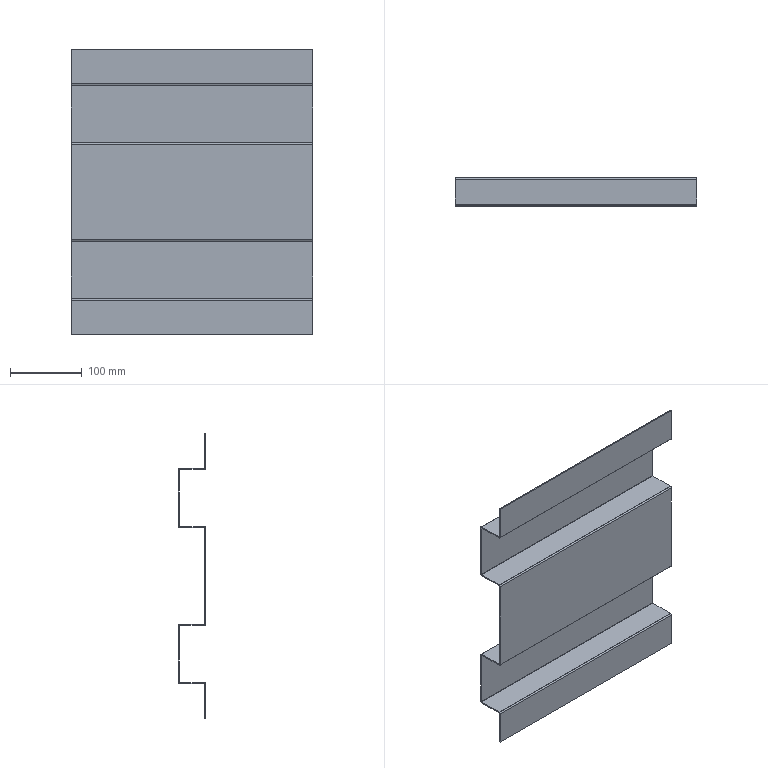Component | SolidWorks | dbj3-1_w14-1 | 1 solid | 70 faces | volume 273328 mm3 | plane 54 | cylinder 16 | commonest cylinder face diameters 4 x8 1 x8